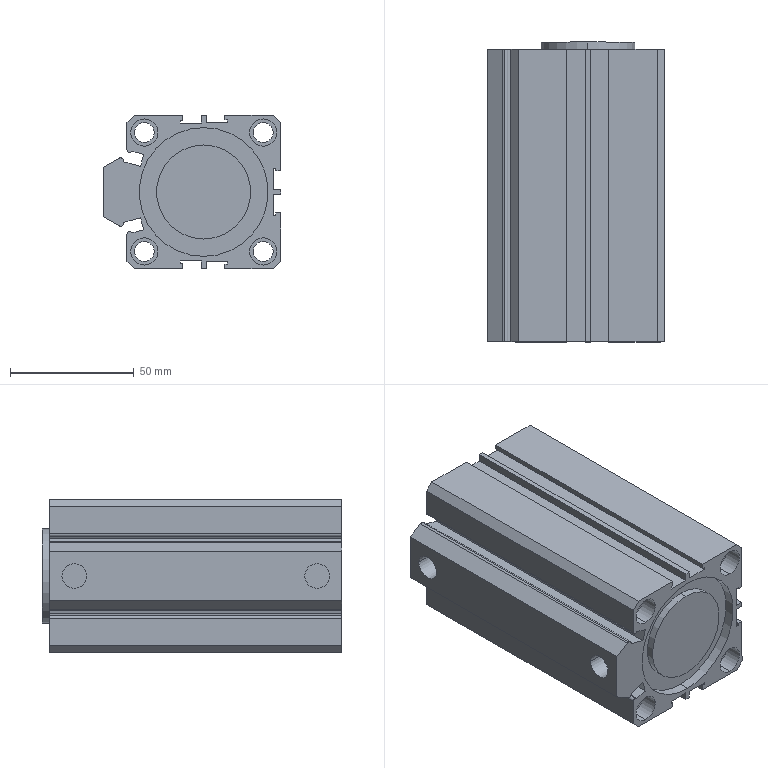Component | SolidWorks | SDA50-80Cylinder-1 | 1 solid | 115 faces | box 71.5 x 121 x 62 mm | volume 399359 mm3 | plane 71 | cylinder 44 | commonest cylinder face diameters 11 x16 8 x8 10 x4 38 x4 52 x4 2.057 x3 2.687 x3 20 x2
build123d program:
from build123d import *

# Parameters (mm, degrees)
BOSS_EXTRUDE1_DEPTH = 118
SKETCH2_R           = 26
CUT_EXTRUDE1_DEPTH  = 4
SKETCH3_R           = 19
BOSS_EXTRUDE2_DEPTH = 3
SKETCH4_R           = 26
CUT_EXTRUDE2_DEPTH  = 4
SKETCH5_R           = 19
BOSS_EXTRUDE3_DEPTH = 7
SKETCH6_R           = 10
CUT_EXTRUDE3_DEPTH  = 70
SKETCH7_R           = 4
CUT_EXTRUDE4_DEPTH  = 246.609
SKETCH8_R           = 5.5
CUT_EXTRUDE5_DEPTH  = 7
CUT_EXTRUDE6_START  = -7
SKETCH9_R           = 5.5
CUT_EXTRUDE6_DEPTH  = 7
SKETCH10_R          = 5
CUT_EXTRUDE7_DEPTH  = 10
CHAMFER1_SIZE       = 3


with BuildPart() as part:
    # Sketch1 → Boss-Extrude1 (new body)
    with BuildSketch(Plane.XY):
        with BuildLine():
            Line((160.374, 76.472), (180.374, 76.472))
            Line((180.374, 76.472), (183.874, 70.41))
            ThreePointArc((183.874, 70.41), (183.976, 68.892), (182.596, 68.252))
            Line((182.596, 68.252), (180.784, 61.491))
            Line((180.784, 61.491), (185.614, 60.197))
            Line((185.614, 60.197), (186.908, 65.026))
            ThreePointArc((186.908, 65.026), (186.374, 66.183), (187.374, 66.972))
            Line((187.374, 66.972), (201.374, 66.972))
            Line((201.374, 66.972), (201.374, 44.413))
            Line((201.374, 44.413), (199.301, 44.413))
            Line((199.301, 44.413), (199.301, 45.475))
            Line((199.301, 45.475), (198.187, 45.475))
            Line((198.187, 45.475), (198.187, 36.991))
            Line((198.187, 36.991), (201.374, 36.991))
            Line((201.374, 36.991), (201.374, 34.954))
            Line((201.374, 34.954), (198.45, 34.954))
            Line((198.45, 34.954), (198.45, 26.475))
            Line((198.45, 26.475), (199.45, 26.475))
            Line((199.45, 26.475), (199.45, 27.475))
            Line((199.45, 27.475), (201.374, 27.475))
            Line((201.374, 27.475), (201.374, 4.972))
            Line((201.374, 4.972), (178.781, 4.972))
            Line((178.781, 4.972), (178.781, 6.992))
            Line((178.781, 6.992), (179.874, 6.992))
            Line((179.874, 6.992), (179.873, 7.992))
            Line((179.873, 7.992), (171.374, 7.99))
            Line((171.374, 7.99), (171.374, 4.972))
            Line((171.374, 4.972), (169.374, 4.972))
            Line((169.374, 4.972), (169.374, 7.989))
            Line((169.374, 7.989), (160.873, 7.986))
            Line((160.873, 7.986), (160.874, 6.986))
            Line((160.874, 6.986), (161.781, 6.987))
            Line((161.781, 6.987), (161.781, 4.972))
            Line((161.781, 4.972), (139.374, 4.972))
            Line((139.374, 4.972), (139.374, 27.475))
            Line((139.374, 27.475), (141.299, 27.475))
            Line((141.299, 27.475), (141.299, 26.475))
            Line((141.299, 26.475), (142.299, 26.475))
            Line((142.299, 26.475), (142.299, 34.954))
            Line((142.299, 34.954), (139.374, 34.954))
            Line((139.374, 34.954), (139.374, 36.991))
            Line((139.374, 36.991), (142.562, 36.991))
            Line((142.562, 36.991), (142.562, 45.475))
            Line((142.562, 45.475), (141.448, 45.475))
            Line((141.448, 45.475), (141.448, 44.413))
            Line((141.448, 44.413), (139.374, 44.413))
            Line((139.374, 44.413), (139.374, 66.972))
            Line((139.374, 66.972), (153.42, 66.972))
            ThreePointArc((153.42, 66.972), (154.42, 66.183), (153.886, 65.026))
            Line((153.886, 65.026), (155.18, 60.197))
            Line((155.18, 60.197), (160.01, 61.491))
            Line((160.01, 61.491), (158.198, 68.252))
            ThreePointArc((158.198, 68.252), (156.776, 68.864), (156.874, 70.41))
            Line((156.874, 70.41), (160.374, 76.472))
        make_face()
    extrude(amount=BOSS_EXTRUDE1_DEPTH)

    # Sketch2 → Cut-Extrude1 (cut)
    with BuildSketch(Plane(origin=(0, 0, 0), x_dir=(-1, 0, 0), z_dir=(0, 0, -1))):
        with Locations((-170.374, 36.001)):
            Circle(SKETCH2_R)
    extrude(amount=-CUT_EXTRUDE1_DEPTH, mode=Mode.SUBTRACT)

    # Sketch3 → Boss-Extrude2 (add)
    with BuildSketch(Plane(origin=(0, 0, 4), x_dir=(-1, 0, 0), z_dir=(0, 0, -1))):
        with Locations((-170.374, 36.001)):
            Circle(SKETCH3_R)
    extrude(amount=BOSS_EXTRUDE2_DEPTH)

    # Sketch4 → Cut-Extrude2 (cut)
    with BuildSketch(Plane.XY.offset(118)):
        with Locations((170.374, 35.972)):
            Circle(SKETCH4_R)
    extrude(amount=-CUT_EXTRUDE2_DEPTH, mode=Mode.SUBTRACT)

    # Sketch5 → Boss-Extrude3 (add)
    with BuildSketch(Plane.XY.offset(114)):
        with Locations((170.374, 35.972)):
            Circle(SKETCH5_R)
    extrude(amount=BOSS_EXTRUDE3_DEPTH)

    # Sketch6 → Cut-Extrude3 (cut)
    with BuildSketch(Plane.XY.offset(121)):
        with Locations((170.374, 35.972)):
            Circle(SKETCH6_R)
    extrude(amount=-CUT_EXTRUDE3_DEPTH, mode=Mode.SUBTRACT)

    # Sketch7 → Cut-Extrude4 (cut, through all)
    with BuildSketch(Plane.XY.offset(118)):
        with Locations((146.374, 59.972)):
            Circle(SKETCH7_R)
        with Locations(Location((194.374, 59.972, 0), (0, 0, 180))):
            Circle(SKETCH7_R)
        with Locations((194.374, 11.972)):
            Circle(SKETCH7_R)
        with Locations(Location((146.374, 11.972, 0), (0, 0, 180))):
            Circle(SKETCH7_R)
    extrude(amount=-CUT_EXTRUDE4_DEPTH, mode=Mode.SUBTRACT)

    # Sketch8 → Cut-Extrude5 (cut)
    with BuildSketch(Plane.XY.offset(118)):
        with Locations((146.374, 59.972)):
            Circle(SKETCH8_R)
        with Locations((194.374, 59.972)):
            Circle(SKETCH8_R)
        with Locations((194.374, 11.972)):
            Circle(SKETCH8_R)
        with Locations((146.374, 11.972)):
            Circle(SKETCH8_R)
    extrude(amount=-CUT_EXTRUDE5_DEPTH, mode=Mode.SUBTRACT)

    # Sketch9 → Cut-Extrude6 (cut)
    with BuildSketch(Plane(origin=(0, 0, 0), x_dir=(-1, 0, 0), z_dir=(0, 0, -1)).offset(CUT_EXTRUDE6_START)):
        with Locations(Location((-194.374, 59.972, 0), (0, 0, 180))):
            Circle(SKETCH9_R)
        with Locations(Location((-146.374, 59.972, 0), (0, 0, 180))):
            Circle(SKETCH9_R)
        with Locations(Location((-194.374, 11.972, 0), (0, 0, 180))):
            Circle(SKETCH9_R)
        with Locations(Location((-146.374, 11.972, 0), (0, 0, 180))):
            Circle(SKETCH9_R)
    extrude(amount=CUT_EXTRUDE6_DEPTH, mode=Mode.SUBTRACT)

    # Sketch10 → Cut-Extrude7 (cut)
    with BuildSketch(Plane(origin=(0, 76.472, 0), x_dir=(1, 0, 0), z_dir=(0, 1, 0))):
        with Locations(Location((170.374, -10, 0), (0, 0, 270))):
            Circle(SKETCH10_R)
        with Locations(Location((170.374, -108, 0), (0, 0, 270))):
            Circle(SKETCH10_R)
    extrude(amount=-CUT_EXTRUDE7_DEPTH, mode=Mode.SUBTRACT)

    # Chamfer1
    chamfer1_edges = [part.edges().sort_by_distance(p)[0] for p in [
        (201.374, 66.972, 59),
        (201.374, 4.972, 59),
        (139.374, 4.972, 59),
        (139.374, 66.972, 59),
    ]]
    chamfer(chamfer1_edges, length=CHAMFER1_SIZE)


solid = part.part

# Placed as in the assembly
solid = solid.moved(Location((6.465, -256.411, 600.874), (-90, 0, 90)))